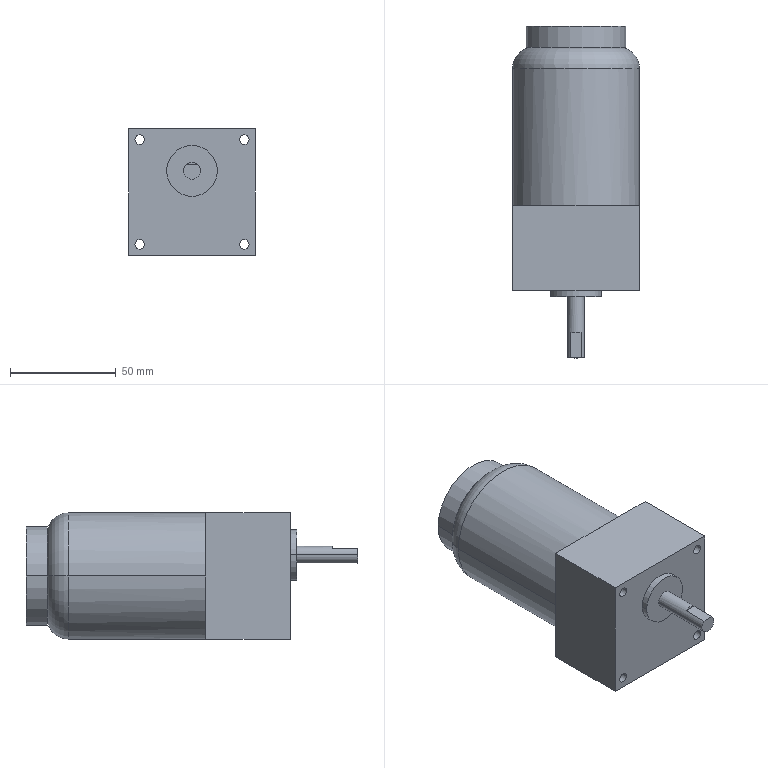Component | SolidWorks | Motor2IK6GN-C-1 | 1 solid | 33 faces | box 60 x 157 x 60 mm | volume 369890 mm3 | cylinder 16 | plane 15 | torus 2 | commonest cylinder face diameters 4.5 x8 47 x2 8 x2 24 x2 60 x2
build123d program:
from build123d import *

# Parameters (mm, degrees)
SKETCH1_W           = 60
SKETCH1_H           = 60
BOSS_EXTRUDE1_DEPTH = 40
SKETCH2_R           = 30
BOSS_EXTRUDE2_DEPTH = 75
FILLET1_R           = 10
SKETCH3_R           = 4
BOSS_EXTRUDE3_DEPTH = 32
SKETCH4_R           = 12
BOSS_EXTRUDE4_DEPTH = 3
CUT_EXTRUDE1_REACH  = 124.577
SKETCH5_R           = 2.25
SKETCH6_W           = 10.613
SKETCH6_H           = 3.192
CUT_EXTRUDE2_DEPTH  = 12
SKETCH7_R           = 23.5
BOSS_EXTRUDE5_DEPTH = 10


with BuildPart() as part:
    # Sketch1 → Boss-Extrude1 (new body)
    with BuildSketch(Plane.XY):
        Rectangle(SKETCH1_W, SKETCH1_H)
    extrude(amount=BOSS_EXTRUDE1_DEPTH)

    # Sketch2 → Boss-Extrude2 (add)
    with BuildSketch(Plane.XY.offset(40)):
        Circle(SKETCH2_R)
    extrude(amount=BOSS_EXTRUDE2_DEPTH)

    # Fillet1
    fillet1_edges = [part.edges().sort_by_distance(p)[0] for p in [
        (-30, 0, 115),
    ]]
    fillet(fillet1_edges, radius=FILLET1_R)

    # Sketch3 → Boss-Extrude3 (add)
    with BuildSketch(Plane(origin=(0, 0, 0), x_dir=(-1, 0, 0), z_dir=(0, 0, -1))):
        with Locations(Location((0, 10, 0), (0, 0, 180))):
            Circle(SKETCH3_R)
    extrude(amount=BOSS_EXTRUDE3_DEPTH)

    # Sketch4 → Boss-Extrude4 (add)
    with BuildSketch(Plane(origin=(0, 0, 0), x_dir=(-1, 0, 0), z_dir=(0, 0, -1))):
        with Locations(Location((0, 10, 0), (0, 0, 180))):
            Circle(SKETCH4_R)
    extrude(amount=BOSS_EXTRUDE4_DEPTH)

    # Sketch5 → Cut-Extrude1 (cut, up to next)
    with BuildSketch(Plane(origin=(0, 0, 0), x_dir=(-1, 0, 0), z_dir=(0, 0, -1)), mode=Mode.PRIVATE) as cut_extrude1_sk1:
        with Locations((-24.75, 24.75)):
            Circle(SKETCH5_R)
    cut_extrude1_tool1 = extrude(cut_extrude1_sk1.sketch, amount=-CUT_EXTRUDE1_REACH, mode=Mode.PRIVATE) & part.part
    # Sketch5 → Cut-Extrude1 (cut, up to next)
    with BuildSketch(Plane(origin=(0, 0, 0), x_dir=(-1, 0, 0), z_dir=(0, 0, -1)), mode=Mode.PRIVATE) as cut_extrude1_sk2:
        with Locations((24.75, 24.75)):
            Circle(SKETCH5_R)
    cut_extrude1_tool2 = extrude(cut_extrude1_sk2.sketch, amount=-CUT_EXTRUDE1_REACH, mode=Mode.PRIVATE) & part.part
    # Sketch5 → Cut-Extrude1 (cut, up to next)
    with BuildSketch(Plane(origin=(0, 0, 0), x_dir=(-1, 0, 0), z_dir=(0, 0, -1)), mode=Mode.PRIVATE) as cut_extrude1_sk3:
        with Locations((-24.75, -24.75)):
            Circle(SKETCH5_R)
    cut_extrude1_tool3 = extrude(cut_extrude1_sk3.sketch, amount=-CUT_EXTRUDE1_REACH, mode=Mode.PRIVATE) & part.part
    # Sketch5 → Cut-Extrude1 (cut, up to next)
    with BuildSketch(Plane(origin=(0, 0, 0), x_dir=(-1, 0, 0), z_dir=(0, 0, -1)), mode=Mode.PRIVATE) as cut_extrude1_sk4:
        with Locations((24.75, -24.75)):
            Circle(SKETCH5_R)
    cut_extrude1_tool4 = extrude(cut_extrude1_sk4.sketch, amount=-CUT_EXTRUDE1_REACH, mode=Mode.PRIVATE) & part.part
    add(cut_extrude1_tool1.solids().sort_by_distance((24.75, 24.75, 0))[0], mode=Mode.SUBTRACT)
    add(cut_extrude1_tool2.solids().sort_by_distance((-24.75, 24.75, 0))[0], mode=Mode.SUBTRACT)
    add(cut_extrude1_tool3.solids().sort_by_distance((24.75, -24.75, 0))[0], mode=Mode.SUBTRACT)
    add(cut_extrude1_tool4.solids().sort_by_distance((-24.75, -24.75, 0))[0], mode=Mode.SUBTRACT)

    # Sketch6 → Cut-Extrude2 (cut)
    with BuildSketch(Plane(origin=(0, 0, -32), x_dir=(-1, 0, 0), z_dir=(0, 0, -1))):
        with Locations((-0.09856, 14.596)):
            Rectangle(SKETCH6_W, SKETCH6_H)
    extrude(amount=-CUT_EXTRUDE2_DEPTH, mode=Mode.SUBTRACT)

    # Sketch7 → Boss-Extrude5 (add)
    with BuildSketch(Plane.XY.offset(115)):
        Circle(SKETCH7_R)
    extrude(amount=BOSS_EXTRUDE5_DEPTH)


solid = part.part

# Placed as in the assembly
solid = solid.moved(Location((-48.547, 10.46, 318), (-90, 0, 180)))
STEP:
#1=COLOUR_RGB('',0.7922,0.8196,0.9333);
#2=FILL_AREA_STYLE_COLOUR('',#1);
#3=FILL_AREA_STYLE('',(#2));
#4=SURFACE_STYLE_FILL_AREA(#3);
#5=SURFACE_SIDE_STYLE('',(#4));
#6=SURFACE_STYLE_USAGE(.BOTH.,#5);
#7=PRESENTATION_STYLE_ASSIGNMENT((#6));
#8=CARTESIAN_POINT('',(-2.837,5.333,12.52));
#9=VERTEX_POINT('',#8);
#10=CARTESIAN_POINT('',(-0.9861,5.333,12.52));
#11=VERTEX_POINT('',#10);
#12=CARTESIAN_POINT('',(-1.911,5.333,12.52));
#13=DIRECTION('',(-0.,1.,-0.));
#14=DIRECTION('',(-1.,0.,0.));
#15=AXIS2_PLACEMENT_3D('',#12,#13,#14);
#16=CIRCLE('',#15,0.9252);
#17=EDGE_CURVE('',#9,#11,#16,.T.);
#18=ORIENTED_EDGE('',*,*,#17,.F.);
#19=CARTESIAN_POINT('',(-2.837,4.939,12.52));
#20=VERTEX_POINT('',#19);
#21=CARTESIAN_POINT('',(-2.837,5.333,12.52));
#22=DIRECTION('',(0.,-1.,0.));
#23=VECTOR('',#22,39.37);
#24=LINE('',#21,#23);
#25=EDGE_CURVE('',#9,#20,#24,.T.);
#26=ORIENTED_EDGE('',*,*,#25,.T.);
#27=CARTESIAN_POINT('',(-0.9861,4.939,12.52));
#28=VERTEX_POINT('',#27);
#29=CARTESIAN_POINT('',(-1.911,4.939,12.52));
#30=DIRECTION('',(-0.,1.,-0.));
#31=DIRECTION('',(-1.,0.,0.));
#32=AXIS2_PLACEMENT_3D('',#29,#30,#31);
#33=CIRCLE('',#32,0.9252);
#34=EDGE_CURVE('',#20,#28,#33,.T.);
#35=ORIENTED_EDGE('',*,*,#34,.T.);
#36=CARTESIAN_POINT('',(-0.9861,5.333,12.52));
#37=DIRECTION('',(0.,-1.,0.));
#38=VECTOR('',#37,39.37);
#39=LINE('',#36,#38);
#40=EDGE_CURVE('',#11,#28,#39,.T.);
#41=ORIENTED_EDGE('',*,*,#40,.F.);
#42=EDGE_LOOP('',(#18,#26,#35,#41));
#43=FACE_OUTER_BOUND('',#42,.T.);
#44=CARTESIAN_POINT('',(-1.911,5.333,12.52));
#45=DIRECTION('',(0.,-1.,0.));
#46=DIRECTION('',(1.,0.,-0.));
#47=AXIS2_PLACEMENT_3D('',#44,#45,#46);
#48=CYLINDRICAL_SURFACE('',#47,0.9252);
#49=ADVANCED_FACE('',(#43),#48,.T.);
#50=CARTESIAN_POINT('',(-1.025,1.987,11.545));
#51=VERTEX_POINT('',#50);
#52=CARTESIAN_POINT('',(-0.8483,1.987,11.545));
#53=VERTEX_POINT('',#52);
#54=CARTESIAN_POINT('',(-0.9369,1.987,11.545));
#55=DIRECTION('',(0.,-1.,0.));
#56=DIRECTION('',(-1.,0.,0.));
#57=AXIS2_PLACEMENT_3D('',#54,#55,#56);
#58=CIRCLE('',#57,0.08858);
#59=EDGE_CURVE('',#51,#53,#58,.T.);
#60=ORIENTED_EDGE('',*,*,#59,.F.);
#61=CARTESIAN_POINT('',(-1.025,0.4118,11.545));
#62=VERTEX_POINT('',#61);
#63=CARTESIAN_POINT('',(-1.025,4.939,11.545));
#64=DIRECTION('',(0.,-1.,0.));
#65=VECTOR('',#64,39.37);
#66=LINE('',#63,#65);
#67=EDGE_CURVE('',#51,#62,#66,.T.);
#68=ORIENTED_EDGE('',*,*,#67,.T.);
#69=CARTESIAN_POINT('',(-0.8483,0.4118,11.545));
#70=VERTEX_POINT('',#69);
#71=CARTESIAN_POINT('',(-0.9369,0.4118,11.545));
#72=DIRECTION('',(0.,-1.,0.));
#73=DIRECTION('',(1.,0.,0.));
#74=AXIS2_PLACEMENT_3D('',#71,#72,#73);
#75=CIRCLE('',#74,0.08858);
#76=EDGE_CURVE('',#62,#70,#75,.T.);
#77=ORIENTED_EDGE('',*,*,#76,.T.);
#78=CARTESIAN_POINT('',(-0.8483,4.939,11.545));
#79=DIRECTION('',(0.,-1.,0.));
#80=VECTOR('',#79,39.37);
#81=LINE('',#78,#80);
#82=EDGE_CURVE('',#53,#70,#81,.T.);
#83=ORIENTED_EDGE('',*,*,#82,.F.);
#84=EDGE_LOOP('',(#60,#68,#77,#83));
#85=FACE_OUTER_BOUND('',#84,.T.);
#86=CARTESIAN_POINT('',(-0.9369,4.939,11.545));
#87=DIRECTION('',(0.,-1.,0.));
#88=DIRECTION('',(1.,0.,0.));
#89=AXIS2_PLACEMENT_3D('',#86,#87,#88);
#90=CYLINDRICAL_SURFACE('',#89,0.08858);
#91=ADVANCED_FACE('',(#85),#90,.F.);
#92=CARTESIAN_POINT('',(-2.974,1.987,11.545));
#93=VERTEX_POINT('',#92);
#94=CARTESIAN_POINT('',(-2.797,1.987,11.545));
#95=VERTEX_POINT('',#94);
#96=CARTESIAN_POINT('',(-2.886,1.987,11.545));
#97=DIRECTION('',(0.,-1.,0.));
#98=DIRECTION('',(-1.,0.,0.));
#99=AXIS2_PLACEMENT_3D('',#96,#97,#98);
#100=CIRCLE('',#99,0.08858);
#101=EDGE_CURVE('',#93,#95,#100,.T.);
#102=ORIENTED_EDGE('',*,*,#101,.F.);
#103=CARTESIAN_POINT('',(-2.974,0.4118,11.545));
#104=VERTEX_POINT('',#103);
#105=CARTESIAN_POINT('',(-2.974,4.939,11.545));
#106=DIRECTION('',(0.,-1.,0.));
#107=VECTOR('',#106,39.37);
#108=LINE('',#105,#107);
#109=EDGE_CURVE('',#93,#104,#108,.T.);
#110=ORIENTED_EDGE('',*,*,#109,.T.);
#111=CARTESIAN_POINT('',(-2.797,0.4118,11.545));
#112=VERTEX_POINT('',#111);
#113=CARTESIAN_POINT('',(-2.886,0.4118,11.545));
#114=DIRECTION('',(0.,-1.,0.));
#115=DIRECTION('',(1.,0.,0.));
#116=AXIS2_PLACEMENT_3D('',#113,#114,#115);
#117=CIRCLE('',#116,0.08858);
#118=EDGE_CURVE('',#104,#112,#117,.T.);
#119=ORIENTED_EDGE('',*,*,#118,.T.);
#120=CARTESIAN_POINT('',(-2.797,4.939,11.545));
#121=DIRECTION('',(0.,-1.,0.));
#122=VECTOR('',#121,39.37);
#123=LINE('',#120,#122);
#124=EDGE_CURVE('',#95,#112,#123,.T.);
#125=ORIENTED_EDGE('',*,*,#124,.F.);
#126=EDGE_LOOP('',(#102,#110,#119,#125));
#127=FACE_OUTER_BOUND('',#126,.T.);
#128=CARTESIAN_POINT('',(-2.886,4.939,11.545));
#129=DIRECTION('',(0.,-1.,0.));
#130=DIRECTION('',(1.,0.,0.));
#131=AXIS2_PLACEMENT_3D('',#128,#129,#130);
#132=CYLINDRICAL_SURFACE('',#131,0.08858);
#133=ADVANCED_FACE('',(#127),#132,.F.);
#134=CARTESIAN_POINT('',(-1.025,1.987,13.494));
#135=VERTEX_POINT('',#134);
#136=CARTESIAN_POINT('',(-0.8483,1.987,13.494));
#137=VERTEX_POINT('',#136);
#138=CARTESIAN_POINT('',(-0.9369,1.987,13.494));
#139=DIRECTION('',(0.,-1.,0.));
#140=DIRECTION('',(-1.,0.,0.));
#141=AXIS2_PLACEMENT_3D('',#138,#139,#140);
#142=CIRCLE('',#141,0.08858);
#143=EDGE_CURVE('',#135,#137,#142,.T.);
#144=ORIENTED_EDGE('',*,*,#143,.F.);
#145=CARTESIAN_POINT('',(-1.025,0.4118,13.494));
#146=VERTEX_POINT('',#145);
#147=CARTESIAN_POINT('',(-1.025,4.939,13.494));
#148=DIRECTION('',(0.,-1.,0.));
#149=VECTOR('',#148,39.37);
#150=LINE('',#147,#149);
#151=EDGE_CURVE('',#135,#146,#150,.T.);
#152=ORIENTED_EDGE('',*,*,#151,.T.);
#153=CARTESIAN_POINT('',(-0.8483,0.4118,13.494));
#154=VERTEX_POINT('',#153);
#155=CARTESIAN_POINT('',(-0.9369,0.4118,13.494));
#156=DIRECTION('',(0.,-1.,0.));
#157=DIRECTION('',(1.,0.,0.));
#158=AXIS2_PLACEMENT_3D('',#155,#156,#157);
#159=CIRCLE('',#158,0.08858);
#160=EDGE_CURVE('',#146,#154,#159,.T.);
#161=ORIENTED_EDGE('',*,*,#160,.T.);
#162=CARTESIAN_POINT('',(-0.8483,4.939,13.494));
#163=DIRECTION('',(0.,-1.,0.));
#164=VECTOR('',#163,39.37);
#165=LINE('',#162,#164);
#166=EDGE_CURVE('',#137,#154,#165,.T.);
#167=ORIENTED_EDGE('',*,*,#166,.F.);
#168=EDGE_LOOP('',(#144,#152,#161,#167));
#169=FACE_OUTER_BOUND('',#168,.T.);
#170=CARTESIAN_POINT('',(-0.9369,4.939,13.494));
#171=DIRECTION('',(0.,-1.,0.));
#172=DIRECTION('',(1.,0.,0.));
#173=AXIS2_PLACEMENT_3D('',#170,#171,#172);
#174=CYLINDRICAL_SURFACE('',#173,0.08858);
#175=ADVANCED_FACE('',(#169),#174,.F.);
#176=CARTESIAN_POINT('',(-2.974,1.987,13.494));
#177=VERTEX_POINT('',#176);
#178=CARTESIAN_POINT('',(-2.797,1.987,13.494));
#179=VERTEX_POINT('',#178);
#180=CARTESIAN_POINT('',(-2.886,1.987,13.494));
#181=DIRECTION('',(0.,-1.,0.));
#182=DIRECTION('',(-1.,0.,0.));
#183=AXIS2_PLACEMENT_3D('',#180,#181,#182);
#184=CIRCLE('',#183,0.08858);
#185=EDGE_CURVE('',#177,#179,#184,.T.);
#186=ORIENTED_EDGE('',*,*,#185,.F.);
#187=CARTESIAN_POINT('',(-2.974,0.4118,13.494));
#188=VERTEX_POINT('',#187);
#189=CARTESIAN_POINT('',(-2.974,4.939,13.494));
#190=DIRECTION('',(0.,-1.,0.));
#191=VECTOR('',#190,39.37);
#192=LINE('',#189,#191);
#193=EDGE_CURVE('',#177,#188,#192,.T.);
#194=ORIENTED_EDGE('',*,*,#193,.T.);
#195=CARTESIAN_POINT('',(-2.797,0.4118,13.494));
#196=VERTEX_POINT('',#195);
#197=CARTESIAN_POINT('',(-2.886,0.4118,13.494));
#198=DIRECTION('',(0.,-1.,0.));
#199=DIRECTION('',(1.,0.,0.));
#200=AXIS2_PLACEMENT_3D('',#197,#198,#199);
#201=CIRCLE('',#200,0.08858);
#202=EDGE_CURVE('',#188,#196,#201,.T.);
#203=ORIENTED_EDGE('',*,*,#202,.T.);
#204=CARTESIAN_POINT('',(-2.797,4.939,13.494));
#205=DIRECTION('',(0.,-1.,0.));
#206=VECTOR('',#205,39.37);
#207=LINE('',#204,#206);
#208=EDGE_CURVE('',#179,#196,#207,.T.);
#209=ORIENTED_EDGE('',*,*,#208,.F.);
#210=EDGE_LOOP('',(#186,#194,#203,#209));
#211=FACE_OUTER_BOUND('',#210,.T.);
#212=CARTESIAN_POINT('',(-2.886,4.939,13.494));
#213=DIRECTION('',(0.,-1.,0.));
#214=DIRECTION('',(1.,0.,0.));
#215=AXIS2_PLACEMENT_3D('',#212,#213,#214);
#216=CYLINDRICAL_SURFACE('',#215,0.08858);
#217=ADVANCED_FACE('',(#211),#216,.F.);
#218=CARTESIAN_POINT('',(-1.754,-0.848,12.913));
#219=VERTEX_POINT('',#218);
#220=CARTESIAN_POINT('',(-1.807,-0.848,13.031));
#221=VERTEX_POINT('',#220);
#222=CARTESIAN_POINT('',(-1.911,-0.848,12.913));
#223=DIRECTION('',(0.,-1.,0.));
#224=DIRECTION('',(1.,0.,-0.));
#225=AXIS2_PLACEMENT_3D('',#222,#223,#224);
#226=CIRCLE('',#225,0.1575);
#227=EDGE_CURVE('',#219,#221,#226,.T.);
#228=ORIENTED_EDGE('',*,*,#227,.F.);
#229=CARTESIAN_POINT('',(-1.754,0.2937,12.913));
#230=VERTEX_POINT('',#229);
#231=CARTESIAN_POINT('',(-1.754,-0.848,12.913));
#232=DIRECTION('',(-0.,1.,-0.));
#233=VECTOR('',#232,39.37);
#234=LINE('',#231,#233);
#235=EDGE_CURVE('',#219,#230,#234,.T.);
#236=ORIENTED_EDGE('',*,*,#235,.T.);
#237=CARTESIAN_POINT('',(-2.069,0.2937,12.913));
#238=VERTEX_POINT('',#237);
#239=CARTESIAN_POINT('',(-1.911,0.2937,12.913));
#240=DIRECTION('',(0.,-1.,0.));
#241=DIRECTION('',(1.,0.,-0.));
#242=AXIS2_PLACEMENT_3D('',#239,#240,#241);
#243=CIRCLE('',#242,0.1575);
#244=EDGE_CURVE('',#230,#238,#243,.T.);
#245=ORIENTED_EDGE('',*,*,#244,.T.);
#246=CARTESIAN_POINT('',(-2.069,-0.848,12.913));
#247=VERTEX_POINT('',#246);
#248=CARTESIAN_POINT('',(-2.069,-0.848,12.913));
#249=DIRECTION('',(-0.,1.,-0.));
#250=VECTOR('',#249,39.37);
#251=LINE('',#248,#250);
#252=EDGE_CURVE('',#247,#238,#251,.T.);
#253=ORIENTED_EDGE('',*,*,#252,.F.);
#254=CARTESIAN_POINT('',(-2.015,-0.848,13.031));
#255=VERTEX_POINT('',#254);
#256=CARTESIAN_POINT('',(-1.911,-0.848,12.913));
#257=DIRECTION('',(0.,-1.,0.));
#258=DIRECTION('',(1.,0.,-0.));
#259=AXIS2_PLACEMENT_3D('',#256,#257,#258);
#260=CIRCLE('',#259,0.1575);
#261=EDGE_CURVE('',#255,#247,#260,.T.);
#262=ORIENTED_EDGE('',*,*,#261,.F.);
#263=CARTESIAN_POINT('',(-2.015,-0.3756,13.031));
#264=VERTEX_POINT('',#263);
#265=CARTESIAN_POINT('',(-2.015,-0.848,13.031));
#266=DIRECTION('',(-0.,1.,-0.));
#267=VECTOR('',#266,39.37);
#268=LINE('',#265,#267);
#269=EDGE_CURVE('',#255,#264,#268,.T.);
#270=ORIENTED_EDGE('',*,*,#269,.T.);
#271=CARTESIAN_POINT('',(-1.807,-0.3756,13.031));
#272=VERTEX_POINT('',#271);
#273=CARTESIAN_POINT('',(-1.911,-0.3756,12.913));
#274=DIRECTION('',(-0.,1.,-0.));
#275=DIRECTION('',(-1.,-0.,0.));
#276=AXIS2_PLACEMENT_3D('',#273,#274,#275);
#277=CIRCLE('',#276,0.1575);
#278=EDGE_CURVE('',#264,#272,#277,.T.);
#279=ORIENTED_EDGE('',*,*,#278,.T.);
#280=CARTESIAN_POINT('',(-1.807,-0.848,13.031));
#281=DIRECTION('',(0.,-1.,0.));
#282=VECTOR('',#281,39.37);
#283=LINE('',#280,#282);
#284=EDGE_CURVE('',#272,#221,#283,.T.);
#285=ORIENTED_EDGE('',*,*,#284,.T.);
#286=EDGE_LOOP('',(#228,#236,#245,#253,#262,#270,#279,#285));
#287=FACE_OUTER_BOUND('',#286,.T.);
#288=CARTESIAN_POINT('',(-1.911,-0.848,12.913));
#289=DIRECTION('',(-0.,1.,-0.));
#290=DIRECTION('',(-1.,-0.,0.));
#291=AXIS2_PLACEMENT_3D('',#288,#289,#290);
#292=CYLINDRICAL_SURFACE('',#291,0.1575);
#293=ADVANCED_FACE('',(#287),#292,.T.);
#294=CARTESIAN_POINT('',(-1.439,0.2937,12.913));
#295=VERTEX_POINT('',#294);
#296=CARTESIAN_POINT('',(-2.384,0.2937,12.913));
#297=VERTEX_POINT('',#296);
#298=CARTESIAN_POINT('',(-1.911,0.2937,12.913));
#299=DIRECTION('',(0.,-1.,0.));
#300=DIRECTION('',(1.,0.,-0.));
#301=AXIS2_PLACEMENT_3D('',#298,#299,#300);
#302=CIRCLE('',#301,0.4724);
#303=EDGE_CURVE('',#295,#297,#302,.T.);
#304=ORIENTED_EDGE('',*,*,#303,.F.);
#305=CARTESIAN_POINT('',(-1.439,0.4118,12.913));
#306=VERTEX_POINT('',#305);
#307=CARTESIAN_POINT('',(-1.439,0.2937,12.913));
#308=DIRECTION('',(-0.,1.,-0.));
#309=VECTOR('',#308,39.37);
#310=LINE('',#307,#309);
#311=EDGE_CURVE('',#295,#306,#310,.T.);
#312=ORIENTED_EDGE('',*,*,#311,.T.);
#313=CARTESIAN_POINT('',(-2.384,0.4118,12.913));
#314=VERTEX_POINT('',#313);
#315=CARTESIAN_POINT('',(-1.911,0.4118,12.913));
#316=DIRECTION('',(0.,-1.,0.));
#317=DIRECTION('',(-1.,-0.,0.));
#318=AXIS2_PLACEMENT_3D('',#315,#316,#317);
#319=CIRCLE('',#318,0.4724);
#320=EDGE_CURVE('',#306,#314,#319,.T.);
#321=ORIENTED_EDGE('',*,*,#320,.T.);
#322=CARTESIAN_POINT('',(-2.384,0.2937,12.913));
#323=DIRECTION('',(-0.,1.,-0.));
#324=VECTOR('',#323,39.37);
#325=LINE('',#322,#324);
#326=EDGE_CURVE('',#297,#314,#325,.T.);
#327=ORIENTED_EDGE('',*,*,#326,.F.);
#328=EDGE_LOOP('',(#304,#312,#321,#327));
#329=FACE_OUTER_BOUND('',#328,.T.);
#330=CARTESIAN_POINT('',(-1.911,0.2937,12.913));
#331=DIRECTION('',(-0.,1.,-0.));
#332=DIRECTION('',(-1.,-0.,0.));
#333=AXIS2_PLACEMENT_3D('',#330,#331,#332);
#334=CYLINDRICAL_SURFACE('',#333,0.4724);
#335=ADVANCED_FACE('',(#329),#334,.T.);
#336=CARTESIAN_POINT('',(-0.7302,4.546,12.52));
#337=VERTEX_POINT('',#336);
#338=CARTESIAN_POINT('',(-3.092,4.546,12.52));
#339=VERTEX_POINT('',#338);
#340=CARTESIAN_POINT('',(-1.911,4.546,12.52));
#341=DIRECTION('',(0.,-1.,0.));
#342=DIRECTION('',(-1.,-0.,0.));
#343=AXIS2_PLACEMENT_3D('',#340,#341,#342);
#344=CIRCLE('',#343,1.181);
#345=EDGE_CURVE('',#337,#339,#344,.T.);
#346=ORIENTED_EDGE('',*,*,#345,.F.);
#347=CARTESIAN_POINT('',(-1.124,4.939,12.52));
#348=VERTEX_POINT('',#347);
#349=CARTESIAN_POINT('',(-1.124,4.546,12.52));
#350=DIRECTION('',(0.,0.,1.));
#351=DIRECTION('',(1.,0.,-0.));
#352=AXIS2_PLACEMENT_3D('',#349,#350,#351);
#353=CIRCLE('',#352,0.3937);
#354=EDGE_CURVE('',#337,#348,#353,.T.);
#355=ORIENTED_EDGE('',*,*,#354,.T.);
#356=CARTESIAN_POINT('',(-2.699,4.939,12.52));
#357=VERTEX_POINT('',#356);
#358=CARTESIAN_POINT('',(-1.911,4.939,12.52));
#359=DIRECTION('',(-0.,1.,-0.));
#360=DIRECTION('',(-1.,0.,0.));
#361=AXIS2_PLACEMENT_3D('',#358,#359,#360);
#362=CIRCLE('',#361,0.7874);
#363=EDGE_CURVE('',#357,#348,#362,.T.);
#364=ORIENTED_EDGE('',*,*,#363,.F.);
#365=CARTESIAN_POINT('',(-2.699,4.546,12.52));
#366=DIRECTION('',(-0.,-0.,-1.));
#367=DIRECTION('',(-1.,0.,0.));
#368=AXIS2_PLACEMENT_3D('',#365,#366,#367);
#369=CIRCLE('',#368,0.3937);
#370=EDGE_CURVE('',#339,#357,#369,.T.);
#371=ORIENTED_EDGE('',*,*,#370,.F.);
#372=EDGE_LOOP('',(#346,#355,#364,#371));
#373=FACE_OUTER_BOUND('',#372,.T.);
#374=CARTESIAN_POINT('',(-1.911,4.546,12.52));
#375=DIRECTION('',(-0.,1.,-0.));
#376=DIRECTION('',(-1.,-0.,0.));
#377=AXIS2_PLACEMENT_3D('',#374,#375,#376);
#378=TOROIDAL_SURFACE('',#377,0.7874,0.3937);
#379=ADVANCED_FACE('',(#373),#378,.T.);
#380=ORIENTED_EDGE('',*,*,#345,.T.);
#381=CARTESIAN_POINT('',(-3.092,1.987,12.52));
#382=VERTEX_POINT('',#381);
#383=CARTESIAN_POINT('',(-3.092,4.939,12.52));
#384=DIRECTION('',(0.,-1.,0.));
#385=VECTOR('',#384,39.37);
#386=LINE('',#383,#385);
#387=EDGE_CURVE('',#339,#382,#386,.T.);
#388=ORIENTED_EDGE('',*,*,#387,.T.);
#389=CARTESIAN_POINT('',(-1.911,1.987,13.701));
#390=VERTEX_POINT('',#389);
#391=CARTESIAN_POINT('',(-1.911,1.987,12.52));
#392=DIRECTION('',(-0.,1.,-0.));
#393=DIRECTION('',(-1.,-0.,0.));
#394=AXIS2_PLACEMENT_3D('',#391,#392,#393);
#395=CIRCLE('',#394,1.181);
#396=EDGE_CURVE('',#382,#390,#395,.T.);
#397=ORIENTED_EDGE('',*,*,#396,.T.);
#398=CARTESIAN_POINT('',(-0.7302,1.987,12.52));
#399=VERTEX_POINT('',#398);
#400=CARTESIAN_POINT('',(-1.911,1.987,12.52));
#401=DIRECTION('',(-0.,1.,-0.));
#402=DIRECTION('',(-1.,-0.,0.));
#403=AXIS2_PLACEMENT_3D('',#400,#401,#402);
#404=CIRCLE('',#403,1.181);
#405=EDGE_CURVE('',#390,#399,#404,.T.);
#406=ORIENTED_EDGE('',*,*,#405,.T.);
#407=CARTESIAN_POINT('',(-0.7302,4.939,12.52));
#408=DIRECTION('',(0.,-1.,0.));
#409=VECTOR('',#408,39.37);
#410=LINE('',#407,#409);
#411=EDGE_CURVE('',#337,#399,#410,.T.);
#412=ORIENTED_EDGE('',*,*,#411,.F.);
#413=EDGE_LOOP('',(#380,#388,#397,#406,#412));
#414=FACE_OUTER_BOUND('',#413,.T.);
#415=CARTESIAN_POINT('',(-1.911,4.939,12.52));
#416=DIRECTION('',(0.,-1.,0.));
#417=DIRECTION('',(1.,0.,-0.));
#418=AXIS2_PLACEMENT_3D('',#415,#416,#417);
#419=CYLINDRICAL_SURFACE('',#418,1.181);
#420=ADVANCED_FACE('',(#414),#419,.T.);
#421=CARTESIAN_POINT('',(-0.9369,0.4118,11.545));
#422=DIRECTION('',(0.,-1.,0.));
#423=DIRECTION('',(1.,0.,0.));
#424=AXIS2_PLACEMENT_3D('',#421,#422,#423);
#425=CIRCLE('',#424,0.08858);
#426=EDGE_CURVE('',#70,#62,#425,.T.);
#427=ORIENTED_EDGE('',*,*,#426,.F.);
#428=ORIENTED_EDGE('',*,*,#76,.F.);
#429=EDGE_LOOP('',(#427,#428));
#430=FACE_BOUND('',#429,.T.);
#431=CARTESIAN_POINT('',(-2.886,0.4118,11.545));
#432=DIRECTION('',(0.,-1.,0.));
#433=DIRECTION('',(1.,0.,0.));
#434=AXIS2_PLACEMENT_3D('',#431,#432,#433);
#435=CIRCLE('',#434,0.08858);
#436=EDGE_CURVE('',#112,#104,#435,.T.);
#437=ORIENTED_EDGE('',*,*,#436,.F.);
#438=ORIENTED_EDGE('',*,*,#118,.F.);
#439=EDGE_LOOP('',(#437,#438));
#440=FACE_BOUND('',#439,.T.);
#441=CARTESIAN_POINT('',(-0.9369,0.4118,13.494));
#442=DIRECTION('',(0.,-1.,0.));
#443=DIRECTION('',(1.,0.,0.));
#444=AXIS2_PLACEMENT_3D('',#441,#442,#443);
#445=CIRCLE('',#444,0.08858);
#446=EDGE_CURVE('',#154,#146,#445,.T.);
#447=ORIENTED_EDGE('',*,*,#446,.F.);
#448=ORIENTED_EDGE('',*,*,#160,.F.);
#449=EDGE_LOOP('',(#447,#448));
#450=FACE_BOUND('',#449,.T.);
#451=CARTESIAN_POINT('',(-2.886,0.4118,13.494));
#452=DIRECTION('',(0.,-1.,0.));
#453=DIRECTION('',(1.,0.,0.));
#454=AXIS2_PLACEMENT_3D('',#451,#452,#453);
#455=CIRCLE('',#454,0.08858);
#456=EDGE_CURVE('',#196,#188,#455,.T.);
#457=ORIENTED_EDGE('',*,*,#456,.F.);
#458=ORIENTED_EDGE('',*,*,#202,.F.);
#459=EDGE_LOOP('',(#457,#458));
#460=FACE_BOUND('',#459,.T.);
#461=CARTESIAN_POINT('',(-0.7302,0.4118,13.701));
#462=VERTEX_POINT('',#461);
#463=CARTESIAN_POINT('',(-0.7302,0.4118,11.339));
#464=VERTEX_POINT('',#463);
#465=CARTESIAN_POINT('',(-0.7302,0.4118,13.701));
#466=DIRECTION('',(-0.,-0.,-1.));
#467=VECTOR('',#466,39.37);
#468=LINE('',#465,#467);
#469=EDGE_CURVE('',#462,#464,#468,.T.);
#470=ORIENTED_EDGE('',*,*,#469,.F.);
#471=CARTESIAN_POINT('',(-3.092,0.4118,13.701));
#472=VERTEX_POINT('',#471);
#473=CARTESIAN_POINT('',(-0.7302,0.4118,13.701));
#474=DIRECTION('',(1.,0.,-0.));
#475=VECTOR('',#474,39.37);
#476=LINE('',#473,#475);
#477=EDGE_CURVE('',#472,#462,#476,.T.);
#478=ORIENTED_EDGE('',*,*,#477,.F.);
#479=CARTESIAN_POINT('',(-3.092,0.4118,11.339));
#480=VERTEX_POINT('',#479);
#481=CARTESIAN_POINT('',(-3.092,0.4118,13.701));
#482=DIRECTION('',(0.,0.,1.));
#483=VECTOR('',#482,39.37);
#484=LINE('',#481,#483);
#485=EDGE_CURVE('',#480,#472,#484,.T.);
#486=ORIENTED_EDGE('',*,*,#485,.F.);
#487=CARTESIAN_POINT('',(-0.7302,0.4118,11.339));
#488=DIRECTION('',(-1.,-0.,0.));
#489=VECTOR('',#488,39.37);
#490=LINE('',#487,#489);
#491=EDGE_CURVE('',#464,#480,#490,.T.);
#492=ORIENTED_EDGE('',*,*,#491,.F.);
#493=EDGE_LOOP('',(#470,#478,#486,#492));
#494=FACE_OUTER_BOUND('',#493,.T.);
#495=CARTESIAN_POINT('',(-1.911,0.4118,12.913));
#496=DIRECTION('',(0.,-1.,0.));
#497=DIRECTION('',(-1.,-0.,0.));
#498=AXIS2_PLACEMENT_3D('',#495,#496,#497);
#499=CIRCLE('',#498,0.4724);
#500=EDGE_CURVE('',#314,#306,#499,.T.);
#501=ORIENTED_EDGE('',*,*,#500,.F.);
#502=ORIENTED_EDGE('',*,*,#320,.F.);
#503=EDGE_LOOP('',(#501,#502));
#504=FACE_BOUND('',#503,.T.);
#505=CARTESIAN_POINT('',(-0.7302,0.4118,11.339));
#506=DIRECTION('',(-0.,1.,-0.));
#507=DIRECTION('',(-1.,-0.,0.));
#508=AXIS2_PLACEMENT_3D('',#505,#506,#507);
#509=PLANE('',#508);
#510=ADVANCED_FACE('',(#430,#440,#450,#460,#494,#504),#509,.F.);
#511=CARTESIAN_POINT('',(-2.886,1.987,13.494));
#512=DIRECTION('',(0.,-1.,0.));
#513=DIRECTION('',(-1.,0.,0.));
#514=AXIS2_PLACEMENT_3D('',#511,#512,#513);
#515=CIRCLE('',#514,0.08858);
#516=EDGE_CURVE('',#179,#177,#515,.T.);
#517=ORIENTED_EDGE('',*,*,#516,.T.);
#518=ORIENTED_EDGE('',*,*,#185,.T.);
#519=EDGE_LOOP('',(#517,#518));
#520=FACE_BOUND('',#519,.T.);
#521=ORIENTED_EDGE('',*,*,#396,.F.);
#522=CARTESIAN_POINT('',(-3.092,1.987,13.701));
#523=VERTEX_POINT('',#522);
#524=CARTESIAN_POINT('',(-3.092,1.987,13.701));
#525=DIRECTION('',(0.,0.,1.));
#526=VECTOR('',#525,39.37);
#527=LINE('',#524,#526);
#528=EDGE_CURVE('',#382,#523,#527,.T.);
#529=ORIENTED_EDGE('',*,*,#528,.T.);
#530=CARTESIAN_POINT('',(-0.7302,1.987,13.701));
#531=DIRECTION('',(1.,0.,-0.));
#532=VECTOR('',#531,39.37);
#533=LINE('',#530,#532);
#534=EDGE_CURVE('',#523,#390,#533,.T.);
#535=ORIENTED_EDGE('',*,*,#534,.T.);
#536=EDGE_LOOP('',(#521,#529,#535));
#537=FACE_OUTER_BOUND('',#536,.T.);
#538=CARTESIAN_POINT('',(-0.7302,1.987,11.339));
#539=DIRECTION('',(-0.,1.,-0.));
#540=DIRECTION('',(-1.,-0.,0.));
#541=AXIS2_PLACEMENT_3D('',#538,#539,#540);
#542=PLANE('',#541);
#543=ADVANCED_FACE('',(#520,#537),#542,.T.);
#544=CARTESIAN_POINT('',(-0.9369,1.987,13.494));
#545=DIRECTION('',(0.,-1.,0.));
#546=DIRECTION('',(-1.,0.,0.));
#547=AXIS2_PLACEMENT_3D('',#544,#545,#546);
#548=CIRCLE('',#547,0.08858);
#549=EDGE_CURVE('',#137,#135,#548,.T.);
#550=ORIENTED_EDGE('',*,*,#549,.T.);
#551=ORIENTED_EDGE('',*,*,#143,.T.);
#552=EDGE_LOOP('',(#550,#551));
#553=FACE_BOUND('',#552,.T.);
#554=ORIENTED_EDGE('',*,*,#405,.F.);
#555=CARTESIAN_POINT('',(-0.7302,1.987,13.701));
#556=VERTEX_POINT('',#555);
#557=CARTESIAN_POINT('',(-0.7302,1.987,13.701));
#558=DIRECTION('',(1.,0.,-0.));
#559=VECTOR('',#558,39.37);
#560=LINE('',#557,#559);
#561=EDGE_CURVE('',#390,#556,#560,.T.);
#562=ORIENTED_EDGE('',*,*,#561,.T.);
#563=CARTESIAN_POINT('',(-0.7302,1.987,13.701));
#564=DIRECTION('',(-0.,-0.,-1.));
#565=VECTOR('',#564,39.37);
#566=LINE('',#563,#565);
#567=EDGE_CURVE('',#556,#399,#566,.T.);
#568=ORIENTED_EDGE('',*,*,#567,.T.);
#569=EDGE_LOOP('',(#554,#562,#568));
#570=FACE_OUTER_BOUND('',#569,.T.);
#571=CARTESIAN_POINT('',(-0.7302,1.987,11.339));
#572=DIRECTION('',(-0.,1.,-0.));
#573=DIRECTION('',(-1.,-0.,0.));
#574=AXIS2_PLACEMENT_3D('',#571,#572,#573);
#575=PLANE('',#574);
#576=ADVANCED_FACE('',(#553,#570),#575,.T.);
#577=CARTESIAN_POINT('',(-0.9369,1.987,11.545));
#578=DIRECTION('',(0.,-1.,0.));
#579=DIRECTION('',(-1.,0.,0.));
#580=AXIS2_PLACEMENT_3D('',#577,#578,#579);
#581=CIRCLE('',#580,0.08858);
#582=EDGE_CURVE('',#53,#51,#581,.T.);
#583=ORIENTED_EDGE('',*,*,#582,.T.);
#584=ORIENTED_EDGE('',*,*,#59,.T.);
#585=EDGE_LOOP('',(#583,#584));
#586=FACE_BOUND('',#585,.T.);
#587=CARTESIAN_POINT('',(-1.911,1.987,11.339));
#588=VERTEX_POINT('',#587);
#589=CARTESIAN_POINT('',(-1.911,1.987,12.52));
#590=DIRECTION('',(-0.,1.,-0.));
#591=DIRECTION('',(-1.,-0.,0.));
#592=AXIS2_PLACEMENT_3D('',#589,#590,#591);
#593=CIRCLE('',#592,1.181);
#594=EDGE_CURVE('',#399,#588,#593,.T.);
#595=ORIENTED_EDGE('',*,*,#594,.F.);
#596=CARTESIAN_POINT('',(-0.7302,1.987,11.339));
#597=VERTEX_POINT('',#596);
#598=CARTESIAN_POINT('',(-0.7302,1.987,13.701));
#599=DIRECTION('',(-0.,-0.,-1.));
#600=VECTOR('',#599,39.37);
#601=LINE('',#598,#600);
#602=EDGE_CURVE('',#399,#597,#601,.T.);
#603=ORIENTED_EDGE('',*,*,#602,.T.);
#604=CARTESIAN_POINT('',(-0.7302,1.987,11.339));
#605=DIRECTION('',(-1.,-0.,0.));
#606=VECTOR('',#605,39.37);
#607=LINE('',#604,#606);
#608=EDGE_CURVE('',#597,#588,#607,.T.);
#609=ORIENTED_EDGE('',*,*,#608,.T.);
#610=EDGE_LOOP('',(#595,#603,#609));
#611=FACE_OUTER_BOUND('',#610,.T.);
#612=CARTESIAN_POINT('',(-0.7302,1.987,11.339));
#613=DIRECTION('',(-0.,1.,-0.));
#614=DIRECTION('',(-1.,-0.,0.));
#615=AXIS2_PLACEMENT_3D('',#612,#613,#614);
#616=PLANE('',#615);
#617=ADVANCED_FACE('',(#586,#611),#616,.T.);
#618=ORIENTED_EDGE('',*,*,#469,.T.);
#619=CARTESIAN_POINT('',(-0.7302,1.987,11.339));
#620=DIRECTION('',(0.,-1.,0.));
#621=VECTOR('',#620,39.37);
#622=LINE('',#619,#621);
#623=EDGE_CURVE('',#597,#464,#622,.T.);
#624=ORIENTED_EDGE('',*,*,#623,.F.);
#625=ORIENTED_EDGE('',*,*,#602,.F.);
#626=ORIENTED_EDGE('',*,*,#567,.F.);
#627=CARTESIAN_POINT('',(-0.7302,1.987,13.701));
#628=DIRECTION('',(0.,-1.,0.));
#629=VECTOR('',#628,39.37);
#630=LINE('',#627,#629);
#631=EDGE_CURVE('',#556,#462,#630,.T.);
#632=ORIENTED_EDGE('',*,*,#631,.T.);
#633=EDGE_LOOP('',(#618,#624,#625,#626,#632));
#634=FACE_OUTER_BOUND('',#633,.T.);
#635=CARTESIAN_POINT('',(-0.7302,1.987,13.701));
#636=DIRECTION('',(-1.,-0.,0.));
#637=DIRECTION('',(0.,-1.,0.));
#638=AXIS2_PLACEMENT_3D('',#635,#636,#637);
#639=PLANE('',#638);
#640=ADVANCED_FACE('',(#634),#639,.F.);
#641=ORIENTED_EDGE('',*,*,#491,.T.);
#642=CARTESIAN_POINT('',(-3.092,1.987,11.339));
#643=VERTEX_POINT('',#642);
#644=CARTESIAN_POINT('',(-3.092,1.987,11.339));
#645=DIRECTION('',(0.,-1.,0.));
#646=VECTOR('',#645,39.37);
#647=LINE('',#644,#646);
#648=EDGE_CURVE('',#643,#480,#647,.T.);
#649=ORIENTED_EDGE('',*,*,#648,.F.);
#650=CARTESIAN_POINT('',(-0.7302,1.987,11.339));
#651=DIRECTION('',(-1.,-0.,0.));
#652=VECTOR('',#651,39.37);
#653=LINE('',#650,#652);
#654=EDGE_CURVE('',#588,#643,#653,.T.);
#655=ORIENTED_EDGE('',*,*,#654,.F.);
#656=ORIENTED_EDGE('',*,*,#608,.F.);
#657=ORIENTED_EDGE('',*,*,#623,.T.);
#658=EDGE_LOOP('',(#641,#649,#655,#656,#657));
#659=FACE_OUTER_BOUND('',#658,.T.);
#660=CARTESIAN_POINT('',(-0.7302,1.987,11.339));
#661=DIRECTION('',(0.,0.,1.));
#662=DIRECTION('',(1.,0.,-0.));
#663=AXIS2_PLACEMENT_3D('',#660,#661,#662);
#664=PLANE('',#663);
#665=ADVANCED_FACE('',(#659),#664,.F.);
#666=ORIENTED_EDGE('',*,*,#485,.T.);
#667=CARTESIAN_POINT('',(-3.092,1.987,13.701));
#668=DIRECTION('',(0.,-1.,0.));
#669=VECTOR('',#668,39.37);
#670=LINE('',#667,#669);
#671=EDGE_CURVE('',#523,#472,#670,.T.);
#672=ORIENTED_EDGE('',*,*,#671,.F.);
#673=ORIENTED_EDGE('',*,*,#528,.F.);
#674=CARTESIAN_POINT('',(-3.092,1.987,13.701));
#675=DIRECTION('',(0.,0.,1.));
#676=VECTOR('',#675,39.37);
#677=LINE('',#674,#676);
#678=EDGE_CURVE('',#643,#382,#677,.T.);
#679=ORIENTED_EDGE('',*,*,#678,.F.);
#680=ORIENTED_EDGE('',*,*,#648,.T.);
#681=EDGE_LOOP('',(#666,#672,#673,#679,#680));
#682=FACE_OUTER_BOUND('',#681,.T.);
#683=CARTESIAN_POINT('',(-3.092,1.987,13.701));
#684=DIRECTION('',(1.,0.,-0.));
#685=DIRECTION('',(-0.,-0.,-1.));
#686=AXIS2_PLACEMENT_3D('',#683,#684,#685);
#687=PLANE('',#686);
#688=ADVANCED_FACE('',(#682),#687,.F.);
#689=ORIENTED_EDGE('',*,*,#477,.T.);
#690=ORIENTED_EDGE('',*,*,#631,.F.);
#691=ORIENTED_EDGE('',*,*,#561,.F.);
#692=ORIENTED_EDGE('',*,*,#534,.F.);
#693=ORIENTED_EDGE('',*,*,#671,.T.);
#694=EDGE_LOOP('',(#689,#690,#691,#692,#693));
#695=FACE_OUTER_BOUND('',#694,.T.);
#696=CARTESIAN_POINT('',(-0.7302,1.987,13.701));
#697=DIRECTION('',(-0.,-0.,-1.));
#698=DIRECTION('',(0.,-1.,0.));
#699=AXIS2_PLACEMENT_3D('',#696,#697,#698);
#700=PLANE('',#699);
#701=ADVANCED_FACE('',(#695),#700,.F.);
#702=CARTESIAN_POINT('',(-2.886,1.987,11.545));
#703=DIRECTION('',(0.,-1.,0.));
#704=DIRECTION('',(-1.,0.,0.));
#705=AXIS2_PLACEMENT_3D('',#702,#703,#704);
#706=CIRCLE('',#705,0.08858);
#707=EDGE_CURVE('',#95,#93,#706,.T.);
#708=ORIENTED_EDGE('',*,*,#707,.T.);
#709=ORIENTED_EDGE('',*,*,#101,.T.);
#710=EDGE_LOOP('',(#708,#709));
#711=FACE_BOUND('',#710,.T.);
#712=CARTESIAN_POINT('',(-1.911,1.987,12.52));
#713=DIRECTION('',(-0.,1.,-0.));
#714=DIRECTION('',(-1.,-0.,0.));
#715=AXIS2_PLACEMENT_3D('',#712,#713,#714);
#716=CIRCLE('',#715,1.181);
#717=EDGE_CURVE('',#588,#382,#716,.T.);
#718=ORIENTED_EDGE('',*,*,#717,.F.);
#719=ORIENTED_EDGE('',*,*,#654,.T.);
#720=ORIENTED_EDGE('',*,*,#678,.T.);
#721=EDGE_LOOP('',(#718,#719,#720));
#722=FACE_OUTER_BOUND('',#721,.T.);
#723=CARTESIAN_POINT('',(-0.7302,1.987,11.339));
#724=DIRECTION('',(-0.,1.,-0.));
#725=DIRECTION('',(-1.,-0.,0.));
#726=AXIS2_PLACEMENT_3D('',#723,#724,#725);
#727=PLANE('',#726);
#728=ADVANCED_FACE('',(#711,#722),#727,.T.);
#729=ORIENTED_EDGE('',*,*,#387,.F.);
#730=CARTESIAN_POINT('',(-1.911,4.546,12.52));
#731=DIRECTION('',(0.,-1.,0.));
#732=DIRECTION('',(-1.,-0.,0.));
#733=AXIS2_PLACEMENT_3D('',#730,#731,#732);
#734=CIRCLE('',#733,1.181);
#735=EDGE_CURVE('',#339,#337,#734,.T.);
#736=ORIENTED_EDGE('',*,*,#735,.T.);
#737=ORIENTED_EDGE('',*,*,#411,.T.);
#738=ORIENTED_EDGE('',*,*,#594,.T.);
#739=ORIENTED_EDGE('',*,*,#717,.T.);
#740=EDGE_LOOP('',(#729,#736,#737,#738,#739));
#741=FACE_OUTER_BOUND('',#740,.T.);
#742=CARTESIAN_POINT('',(-1.911,4.939,12.52));
#743=DIRECTION('',(0.,-1.,0.));
#744=DIRECTION('',(1.,0.,-0.));
#745=AXIS2_PLACEMENT_3D('',#742,#743,#744);
#746=CYLINDRICAL_SURFACE('',#745,1.181);
#747=ADVANCED_FACE('',(#741),#746,.T.);
#748=ORIENTED_EDGE('',*,*,#354,.F.);
#749=ORIENTED_EDGE('',*,*,#735,.F.);
#750=ORIENTED_EDGE('',*,*,#370,.T.);
#751=CARTESIAN_POINT('',(-1.911,4.939,12.52));
#752=DIRECTION('',(-0.,1.,-0.));
#753=DIRECTION('',(-1.,0.,0.));
#754=AXIS2_PLACEMENT_3D('',#751,#752,#753);
#755=CIRCLE('',#754,0.7874);
#756=EDGE_CURVE('',#348,#357,#755,.T.);
#757=ORIENTED_EDGE('',*,*,#756,.F.);
#758=EDGE_LOOP('',(#748,#749,#750,#757));
#759=FACE_OUTER_BOUND('',#758,.T.);
#760=CARTESIAN_POINT('',(-1.911,4.546,12.52));
#761=DIRECTION('',(-0.,1.,-0.));
#762=DIRECTION('',(-1.,-0.,0.));
#763=AXIS2_PLACEMENT_3D('',#760,#761,#762);
#764=TOROIDAL_SURFACE('',#763,0.7874,0.3937);
#765=ADVANCED_FACE('',(#759),#764,.T.);
#766=CARTESIAN_POINT('',(-1.911,0.2937,12.913));
#767=DIRECTION('',(0.,-1.,0.));
#768=DIRECTION('',(1.,0.,-0.));
#769=AXIS2_PLACEMENT_3D('',#766,#767,#768);
#770=CIRCLE('',#769,0.4724);
#771=EDGE_CURVE('',#297,#295,#770,.T.);
#772=ORIENTED_EDGE('',*,*,#771,.T.);
#773=ORIENTED_EDGE('',*,*,#303,.T.);
#774=EDGE_LOOP('',(#772,#773));
#775=FACE_OUTER_BOUND('',#774,.T.);
#776=CARTESIAN_POINT('',(-1.911,0.2937,12.913));
#777=DIRECTION('',(0.,-1.,0.));
#778=DIRECTION('',(1.,0.,-0.));
#779=AXIS2_PLACEMENT_3D('',#776,#777,#778);
#780=CIRCLE('',#779,0.1575);
#781=EDGE_CURVE('',#238,#230,#780,.T.);
#782=ORIENTED_EDGE('',*,*,#781,.F.);
#783=ORIENTED_EDGE('',*,*,#244,.F.);
#784=EDGE_LOOP('',(#782,#783));
#785=FACE_BOUND('',#784,.T.);
#786=CARTESIAN_POINT('',(-1.911,0.2937,12.913));
#787=DIRECTION('',(0.,-1.,0.));
#788=DIRECTION('',(1.,0.,-0.));
#789=AXIS2_PLACEMENT_3D('',#786,#787,#788);
#790=PLANE('',#789);
#791=ADVANCED_FACE('',(#775,#785),#790,.T.);
#792=ORIENTED_EDGE('',*,*,#311,.F.);
#793=ORIENTED_EDGE('',*,*,#771,.F.);
#794=ORIENTED_EDGE('',*,*,#326,.T.);
#795=ORIENTED_EDGE('',*,*,#500,.T.);
#796=EDGE_LOOP('',(#792,#793,#794,#795));
#797=FACE_OUTER_BOUND('',#796,.T.);
#798=CARTESIAN_POINT('',(-1.911,0.2937,12.913));
#799=DIRECTION('',(-0.,1.,-0.));
#800=DIRECTION('',(-1.,-0.,0.));
#801=AXIS2_PLACEMENT_3D('',#798,#799,#800);
#802=CYLINDRICAL_SURFACE('',#801,0.4724);
#803=ADVANCED_FACE('',(#797),#802,.T.);
#804=CARTESIAN_POINT('',(-2.124,-0.848,13.031));
#805=DIRECTION('',(1.,0.,-0.));
#806=VECTOR('',#805,39.37);
#807=LINE('',#804,#806);
#808=EDGE_CURVE('',#255,#221,#807,.T.);
#809=ORIENTED_EDGE('',*,*,#808,.F.);
#810=ORIENTED_EDGE('',*,*,#261,.T.);
#811=CARTESIAN_POINT('',(-1.911,-0.848,12.913));
#812=DIRECTION('',(0.,-1.,0.));
#813=DIRECTION('',(1.,0.,-0.));
#814=AXIS2_PLACEMENT_3D('',#811,#812,#813);
#815=CIRCLE('',#814,0.1575);
#816=EDGE_CURVE('',#247,#219,#815,.T.);
#817=ORIENTED_EDGE('',*,*,#816,.T.);
#818=ORIENTED_EDGE('',*,*,#227,.T.);
#819=EDGE_LOOP('',(#809,#810,#817,#818));
#820=FACE_OUTER_BOUND('',#819,.T.);
#821=CARTESIAN_POINT('',(-1.911,-0.848,12.913));
#822=DIRECTION('',(0.,-1.,0.));
#823=DIRECTION('',(1.,0.,-0.));
#824=AXIS2_PLACEMENT_3D('',#821,#822,#823);
#825=PLANE('',#824);
#826=ADVANCED_FACE('',(#820),#825,.T.);
#827=ORIENTED_EDGE('',*,*,#235,.F.);
#828=ORIENTED_EDGE('',*,*,#816,.F.);
#829=ORIENTED_EDGE('',*,*,#252,.T.);
#830=ORIENTED_EDGE('',*,*,#781,.T.);
#831=EDGE_LOOP('',(#827,#828,#829,#830));
#832=FACE_OUTER_BOUND('',#831,.T.);
#833=CARTESIAN_POINT('',(-1.911,-0.848,12.913));
#834=DIRECTION('',(-0.,1.,-0.));
#835=DIRECTION('',(-1.,-0.,0.));
#836=AXIS2_PLACEMENT_3D('',#833,#834,#835);
#837=CYLINDRICAL_SURFACE('',#836,0.1575);
#838=ADVANCED_FACE('',(#832),#837,.T.);
#839=ORIENTED_EDGE('',*,*,#193,.F.);
#840=ORIENTED_EDGE('',*,*,#516,.F.);
#841=ORIENTED_EDGE('',*,*,#208,.T.);
#842=ORIENTED_EDGE('',*,*,#456,.T.);
#843=EDGE_LOOP('',(#839,#840,#841,#842));
#844=FACE_OUTER_BOUND('',#843,.T.);
#845=CARTESIAN_POINT('',(-2.886,4.939,13.494));
#846=DIRECTION('',(0.,-1.,0.));
#847=DIRECTION('',(1.,0.,0.));
#848=AXIS2_PLACEMENT_3D('',#845,#846,#847);
#849=CYLINDRICAL_SURFACE('',#848,0.08858);
#850=ADVANCED_FACE('',(#844),#849,.F.);
#851=ORIENTED_EDGE('',*,*,#151,.F.);
#852=ORIENTED_EDGE('',*,*,#549,.F.);
#853=ORIENTED_EDGE('',*,*,#166,.T.);
#854=ORIENTED_EDGE('',*,*,#446,.T.);
#855=EDGE_LOOP('',(#851,#852,#853,#854));
#856=FACE_OUTER_BOUND('',#855,.T.);
#857=CARTESIAN_POINT('',(-0.9369,4.939,13.494));
#858=DIRECTION('',(0.,-1.,0.));
#859=DIRECTION('',(1.,0.,0.));
#860=AXIS2_PLACEMENT_3D('',#857,#858,#859);
#861=CYLINDRICAL_SURFACE('',#860,0.08858);
#862=ADVANCED_FACE('',(#856),#861,.F.);
#863=ORIENTED_EDGE('',*,*,#109,.F.);
#864=ORIENTED_EDGE('',*,*,#707,.F.);
#865=ORIENTED_EDGE('',*,*,#124,.T.);
#866=ORIENTED_EDGE('',*,*,#436,.T.);
#867=EDGE_LOOP('',(#863,#864,#865,#866));
#868=FACE_OUTER_BOUND('',#867,.T.);
#869=CARTESIAN_POINT('',(-2.886,4.939,11.545));
#870=DIRECTION('',(0.,-1.,0.));
#871=DIRECTION('',(1.,0.,0.));
#872=AXIS2_PLACEMENT_3D('',#869,#870,#871);
#873=CYLINDRICAL_SURFACE('',#872,0.08858);
#874=ADVANCED_FACE('',(#868),#873,.F.);
#875=ORIENTED_EDGE('',*,*,#67,.F.);
#876=ORIENTED_EDGE('',*,*,#582,.F.);
#877=ORIENTED_EDGE('',*,*,#82,.T.);
#878=ORIENTED_EDGE('',*,*,#426,.T.);
#879=EDGE_LOOP('',(#875,#876,#877,#878));
#880=FACE_OUTER_BOUND('',#879,.T.);
#881=CARTESIAN_POINT('',(-0.9369,4.939,11.545));
#882=DIRECTION('',(0.,-1.,0.));
#883=DIRECTION('',(1.,0.,0.));
#884=AXIS2_PLACEMENT_3D('',#881,#882,#883);
#885=CYLINDRICAL_SURFACE('',#884,0.08858);
#886=ADVANCED_FACE('',(#880),#885,.F.);
#887=ORIENTED_EDGE('',*,*,#808,.T.);
#888=ORIENTED_EDGE('',*,*,#284,.F.);
#889=CARTESIAN_POINT('',(-2.124,-0.3756,13.031));
#890=DIRECTION('',(1.,0.,-0.));
#891=VECTOR('',#890,39.37);
#892=LINE('',#889,#891);
#893=EDGE_CURVE('',#264,#272,#892,.T.);
#894=ORIENTED_EDGE('',*,*,#893,.F.);
#895=ORIENTED_EDGE('',*,*,#269,.F.);
#896=EDGE_LOOP('',(#887,#888,#894,#895));
#897=FACE_OUTER_BOUND('',#896,.T.);
#898=CARTESIAN_POINT('',(-2.124,-0.3756,13.031));
#899=DIRECTION('',(-0.,-0.,-1.));
#900=DIRECTION('',(0.,-1.,0.));
#901=AXIS2_PLACEMENT_3D('',#898,#899,#900);
#902=PLANE('',#901);
#903=ADVANCED_FACE('',(#897),#902,.F.);
#904=ORIENTED_EDGE('',*,*,#893,.T.);
#905=ORIENTED_EDGE('',*,*,#278,.F.);
#906=EDGE_LOOP('',(#904,#905));
#907=FACE_OUTER_BOUND('',#906,.T.);
#908=CARTESIAN_POINT('',(-1.911,-0.3756,12.52));
#909=DIRECTION('',(-0.,1.,-0.));
#910=DIRECTION('',(-1.,-0.,0.));
#911=AXIS2_PLACEMENT_3D('',#908,#909,#910);
#912=PLANE('',#911);
#913=ADVANCED_FACE('',(#907),#912,.F.);
#914=ORIENTED_EDGE('',*,*,#25,.F.);
#915=CARTESIAN_POINT('',(-1.911,5.333,12.52));
#916=DIRECTION('',(-0.,1.,-0.));
#917=DIRECTION('',(-1.,0.,0.));
#918=AXIS2_PLACEMENT_3D('',#915,#916,#917);
#919=CIRCLE('',#918,0.9252);
#920=EDGE_CURVE('',#11,#9,#919,.T.);
#921=ORIENTED_EDGE('',*,*,#920,.F.);
#922=ORIENTED_EDGE('',*,*,#40,.T.);
#923=CARTESIAN_POINT('',(-1.911,4.939,12.52));
#924=DIRECTION('',(-0.,1.,-0.));
#925=DIRECTION('',(-1.,0.,0.));
#926=AXIS2_PLACEMENT_3D('',#923,#924,#925);
#927=CIRCLE('',#926,0.9252);
#928=EDGE_CURVE('',#28,#20,#927,.T.);
#929=ORIENTED_EDGE('',*,*,#928,.T.);
#930=EDGE_LOOP('',(#914,#921,#922,#929));
#931=FACE_OUTER_BOUND('',#930,.T.);
#932=CARTESIAN_POINT('',(-1.911,5.333,12.52));
#933=DIRECTION('',(0.,-1.,0.));
#934=DIRECTION('',(1.,0.,-0.));
#935=AXIS2_PLACEMENT_3D('',#932,#933,#934);
#936=CYLINDRICAL_SURFACE('',#935,0.9252);
#937=ADVANCED_FACE('',(#931),#936,.T.);
#938=ORIENTED_EDGE('',*,*,#920,.T.);
#939=ORIENTED_EDGE('',*,*,#17,.T.);
#940=EDGE_LOOP('',(#938,#939));
#941=FACE_OUTER_BOUND('',#940,.T.);
#942=CARTESIAN_POINT('',(-1.911,5.333,12.52));
#943=DIRECTION('',(-0.,1.,-0.));
#944=DIRECTION('',(-1.,-0.,0.));
#945=AXIS2_PLACEMENT_3D('',#942,#943,#944);
#946=PLANE('',#945);
#947=ADVANCED_FACE('',(#941),#946,.T.);
#948=ORIENTED_EDGE('',*,*,#363,.T.);
#949=ORIENTED_EDGE('',*,*,#756,.T.);
#950=EDGE_LOOP('',(#948,#949));
#951=FACE_BOUND('',#950,.T.);
#952=ORIENTED_EDGE('',*,*,#928,.F.);
#953=ORIENTED_EDGE('',*,*,#34,.F.);
#954=EDGE_LOOP('',(#952,#953));
#955=FACE_OUTER_BOUND('',#954,.T.);
#956=CARTESIAN_POINT('',(-1.911,4.939,12.52));
#957=DIRECTION('',(-0.,1.,-0.));
#958=DIRECTION('',(-1.,-0.,0.));
#959=AXIS2_PLACEMENT_3D('',#956,#957,#958);
#960=PLANE('',#959);
#961=ADVANCED_FACE('',(#951,#955),#960,.F.);
#962=CLOSED_SHELL('',(#49,#91,#133,#175,#217,#293,#335,#379,#420,#510,#543,#576,#617,#640,#665,#688,#701,#728,#747,#765,#791,#803,#826,#838,#850,#862,#874,#886,#903,#913,#937,#947,#961));
#963=MANIFOLD_SOLID_BREP('',#962);
#964=STYLED_ITEM('',(#7),#963);
#965=PRESENTATION_LAYER_ASSIGNMENT('','',(#964));
#966=CARTESIAN_POINT('',(0.,0.,0.));
#967=DIRECTION('',(0.,0.,1.));
#968=DIRECTION('',(1.,0.,0.));
#969=AXIS2_PLACEMENT_3D('',#966,#967,#968);
#970=(LENGTH_UNIT()NAMED_UNIT(*)SI_UNIT($,.METRE.));
#971=LENGTH_MEASURE_WITH_UNIT(LENGTH_MEASURE(0.0254),#970);
#972=DIMENSIONAL_EXPONENTS(1.,0.,0.,0.,0.,0.,0.);
#973=(CONVERSION_BASED_UNIT('',#971)LENGTH_UNIT()NAMED_UNIT(#972));
#974=UNCERTAINTY_MEASURE_WITH_UNIT(LENGTH_MEASURE(0.00001),#973,'','');
#975=(NAMED_UNIT(*)PLANE_ANGLE_UNIT()SI_UNIT($,.RADIAN.));
#976=(NAMED_UNIT(*)SI_UNIT($,.STERADIAN.)SOLID_ANGLE_UNIT());
#977=(GEOMETRIC_REPRESENTATION_CONTEXT(3)GLOBAL_UNCERTAINTY_ASSIGNED_CONTEXT((#974))GLOBAL_UNIT_ASSIGNED_CONTEXT((#973,#975,#976))REPRESENTATION_CONTEXT('',''));
#978=ADVANCED_BREP_SHAPE_REPRESENTATION('',(#963,#969),#977);
#979=(LENGTH_UNIT()NAMED_UNIT(*)SI_UNIT($,.METRE.));
#980=LENGTH_MEASURE_WITH_UNIT(LENGTH_MEASURE(0.0254),#979);
#981=DIMENSIONAL_EXPONENTS(1.,0.,0.,0.,0.,0.,0.);
#982=(CONVERSION_BASED_UNIT('',#980)LENGTH_UNIT()NAMED_UNIT(#981));
#983=UNCERTAINTY_MEASURE_WITH_UNIT(LENGTH_MEASURE(0.00001),#982,'','');
#984=(NAMED_UNIT(*)PLANE_ANGLE_UNIT()SI_UNIT($,.RADIAN.));
#985=(NAMED_UNIT(*)SI_UNIT($,.STERADIAN.)SOLID_ANGLE_UNIT());
#986=(GEOMETRIC_REPRESENTATION_CONTEXT(3)GLOBAL_UNCERTAINTY_ASSIGNED_CONTEXT((#983))GLOBAL_UNIT_ASSIGNED_CONTEXT((#982,#984,#985))REPRESENTATION_CONTEXT('',''));
#987=MECHANICAL_DESIGN_GEOMETRIC_PRESENTATION_REPRESENTATION('',(#964),#986);